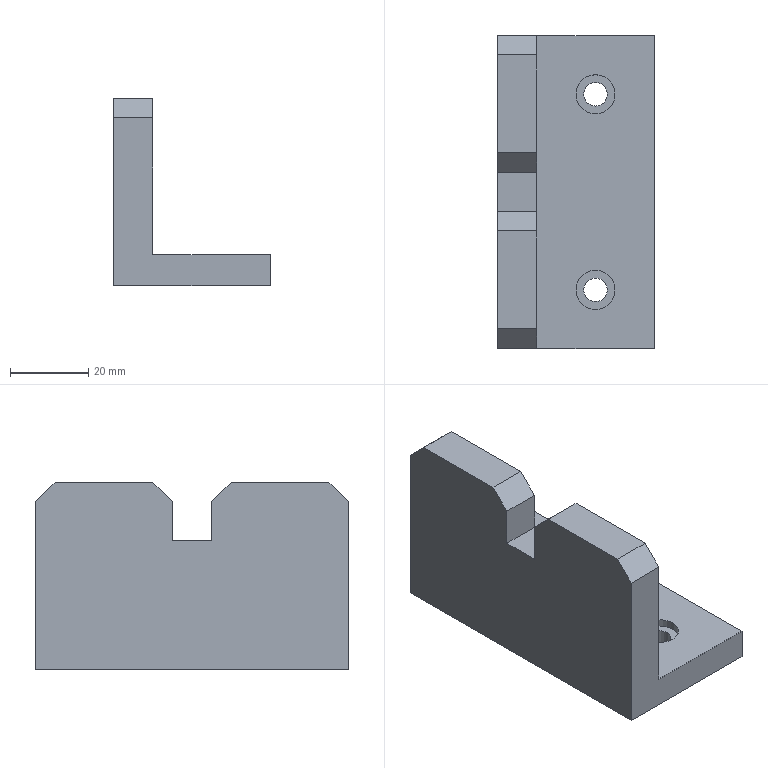Component | NX | 3 | 1 solid | 22 faces | volume 54947 mm3 | plane 18 | cylinder 4 | commonest cylinder face diameters 6 x2 10 x2